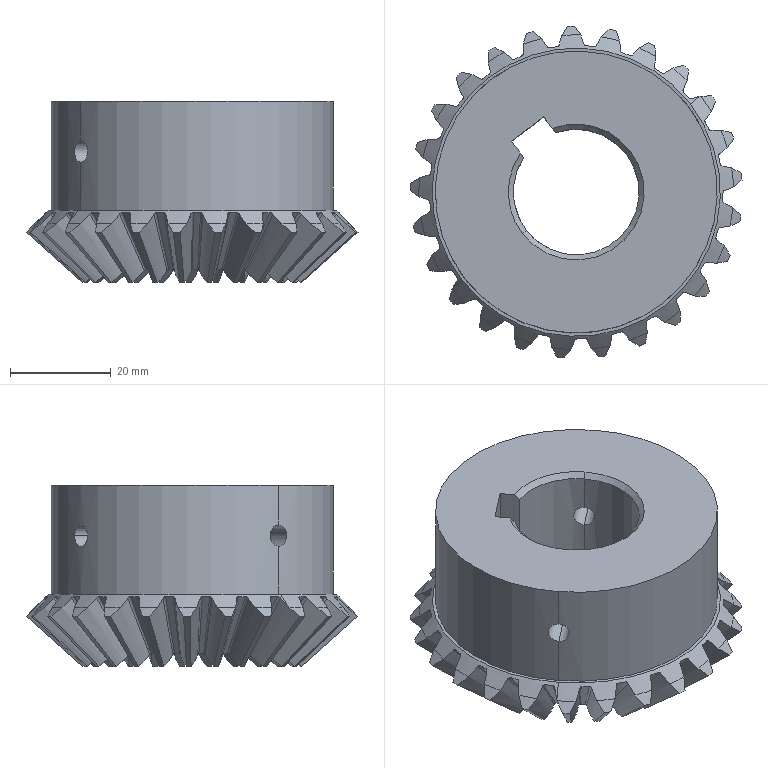Component | SolidWorks | -PullerBevelGear02-2 | 1 solid | 199 faces | volume 62847 mm3 | spline 125 | cone 57 | cylinder 11 | plane 6 | commonest cylinder face diameters 4.2 x6 25 x3 56 x2